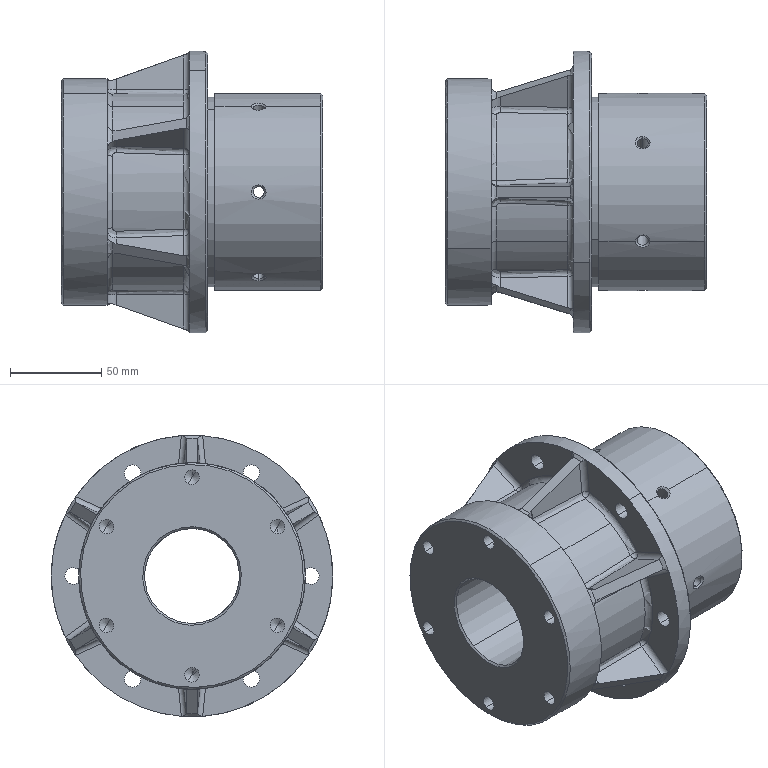Component | SolidWorks | Bushing0718-1 | 1 solid | 237 faces | volume 932547 mm3 | cylinder 97 | plane 38 | spline 35 | cone 34 | torus 18 | sphere 15 | commonest cylinder face diameters 6 x26 10 x22 9 x12 8 x12 108 x9 52 x6 124 x2 154 x2